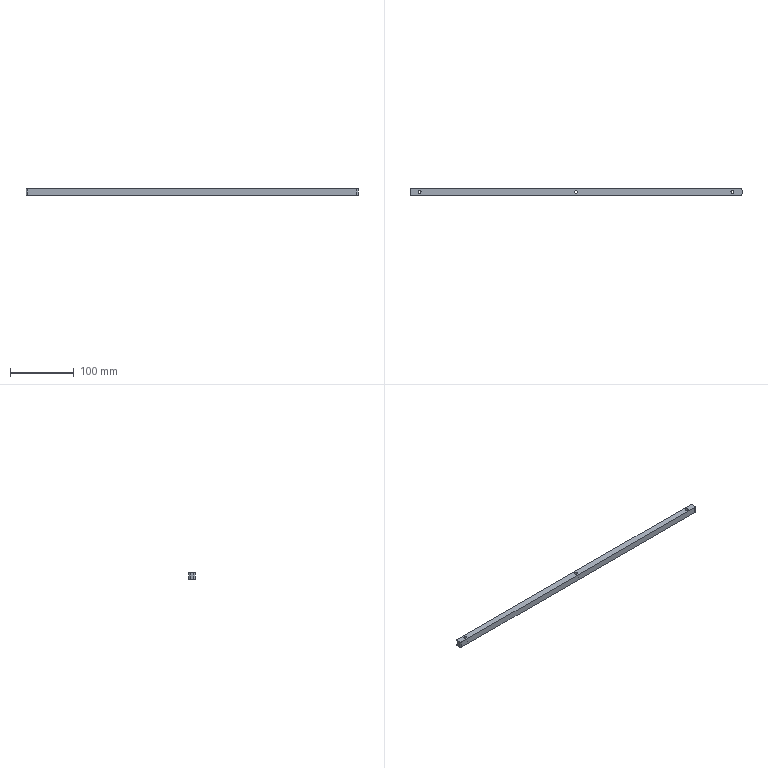Component | SolidWorks | SL010-RightStreamline-1-1_SL010-02047843SupportBar1-1-1 | 1 solid | 25 faces | box 520 x 10 x 10 mm | volume 51035 mm3 | cylinder 16 | plane 9 | commonest cylinder face diameters 8 x6 4.5 x6 4 x4 | material White POM
build123d program:
from build123d import *

# Parameters (mm, degrees)
SKETCH1_W                                       = 520
SKETCH1_H                                       = 10
BOSS_EXTRUDE1_DEPTH                             = 5
M4_HEX_SOCKET_HEAD_CAP_SCREW_CBORE1_D           = 4.5
M4_HEX_SOCKET_HEAD_CAP_SCREW_CBORE1_CBORE_D     = 8
M4_HEX_SOCKET_HEAD_CAP_SCREW_CBORE1_CBORE_DEPTH = 4.4
FILLET1_R                                       = 2


with BuildPart() as part:
    # Sketch1 → Boss-Extrude1 (new, symmetric)
    with BuildSketch(Plane.XY):
        Rectangle(SKETCH1_W, SKETCH1_H)
    extrude(amount=BOSS_EXTRUDE1_DEPTH, both=True)

    # M4 Hex Socket Head Cap Screw CBORE1 (through all)
    with Locations(Plane.XY.offset(5)):
        with Locations((-245, 0), (245, 0), (0, 0)):
            CounterBoreHole(M4_HEX_SOCKET_HEAD_CAP_SCREW_CBORE1_D / 2, M4_HEX_SOCKET_HEAD_CAP_SCREW_CBORE1_CBORE_D / 2, M4_HEX_SOCKET_HEAD_CAP_SCREW_CBORE1_CBORE_DEPTH)

    # Fillet1
    fillet1_edges = [part.edges().sort_by_distance(p)[0] for p in [
        (260, -5, 0),
        (-260, -5, 0),
        (-260, 5, 0),
        (260, 5, 0),
    ]]
    fillet(fillet1_edges, radius=FILLET1_R)


solid = part.part

# Placed as in the assembly
solid = solid.moved(Location((638.47, -116.404, -336.035), (180, 0, 0)))
STEP:
#1=COLOUR_RGB('',0.7922,0.8196,0.9333);
#2=FILL_AREA_STYLE_COLOUR('',#1);
#3=FILL_AREA_STYLE('',(#2));
#4=SURFACE_STYLE_FILL_AREA(#3);
#5=SURFACE_SIDE_STYLE('',(#4));
#6=SURFACE_STYLE_USAGE(.BOTH.,#5);
#7=PRESENTATION_STYLE_ASSIGNMENT((#6));
#8=CARTESIAN_POINT('',(34.94,-4.583,-13.253));
#9=VERTEX_POINT('',#8);
#10=CARTESIAN_POINT('',(34.625,-4.583,-13.253));
#11=VERTEX_POINT('',#10);
#12=CARTESIAN_POINT('',(34.782,-4.583,-13.253));
#13=DIRECTION('',(0.,-0.,-1.));
#14=DIRECTION('',(-1.,0.,0.));
#15=AXIS2_PLACEMENT_3D('',#12,#13,#14);
#16=CIRCLE('',#15,0.1575);
#17=EDGE_CURVE('',#9,#11,#16,.T.);
#18=ORIENTED_EDGE('',*,*,#17,.F.);
#19=CARTESIAN_POINT('',(34.94,-4.583,-13.427));
#20=VERTEX_POINT('',#19);
#21=CARTESIAN_POINT('',(34.94,-4.583,-13.427));
#22=DIRECTION('',(0.,-0.,-1.));
#23=VECTOR('',#22,39.37);
#24=LINE('',#21,#23);
#25=EDGE_CURVE('',#9,#20,#24,.T.);
#26=ORIENTED_EDGE('',*,*,#25,.T.);
#27=CARTESIAN_POINT('',(34.625,-4.583,-13.427));
#28=VERTEX_POINT('',#27);
#29=CARTESIAN_POINT('',(34.782,-4.583,-13.427));
#30=DIRECTION('',(0.,-0.,-1.));
#31=DIRECTION('',(-1.,0.,0.));
#32=AXIS2_PLACEMENT_3D('',#29,#30,#31);
#33=CIRCLE('',#32,0.1575);
#34=EDGE_CURVE('',#20,#28,#33,.T.);
#35=ORIENTED_EDGE('',*,*,#34,.T.);
#36=CARTESIAN_POINT('',(34.625,-4.583,-13.427));
#37=DIRECTION('',(0.,-0.,-1.));
#38=VECTOR('',#37,39.37);
#39=LINE('',#36,#38);
#40=EDGE_CURVE('',#11,#28,#39,.T.);
#41=ORIENTED_EDGE('',*,*,#40,.F.);
#42=EDGE_LOOP('',(#18,#26,#35,#41));
#43=FACE_OUTER_BOUND('',#42,.T.);
#44=CARTESIAN_POINT('',(34.782,-4.583,-13.427));
#45=DIRECTION('',(0.,-0.,-1.));
#46=DIRECTION('',(-1.,0.,0.));
#47=AXIS2_PLACEMENT_3D('',#44,#45,#46);
#48=CYLINDRICAL_SURFACE('',#47,0.1575);
#49=ADVANCED_FACE('',(#43),#48,.F.);
#50=CARTESIAN_POINT('',(34.871,-4.583,-13.033));
#51=VERTEX_POINT('',#50);
#52=CARTESIAN_POINT('',(34.694,-4.583,-13.033));
#53=VERTEX_POINT('',#52);
#54=CARTESIAN_POINT('',(34.782,-4.583,-13.033));
#55=DIRECTION('',(0.,-0.,-1.));
#56=DIRECTION('',(-1.,0.,0.));
#57=AXIS2_PLACEMENT_3D('',#54,#55,#56);
#58=CIRCLE('',#57,0.08858);
#59=EDGE_CURVE('',#51,#53,#58,.T.);
#60=ORIENTED_EDGE('',*,*,#59,.F.);
#61=CARTESIAN_POINT('',(34.871,-4.583,-13.253));
#62=VERTEX_POINT('',#61);
#63=CARTESIAN_POINT('',(34.871,-4.583,-13.427));
#64=DIRECTION('',(0.,-0.,-1.));
#65=VECTOR('',#64,39.37);
#66=LINE('',#63,#65);
#67=EDGE_CURVE('',#51,#62,#66,.T.);
#68=ORIENTED_EDGE('',*,*,#67,.T.);
#69=CARTESIAN_POINT('',(34.694,-4.583,-13.253));
#70=VERTEX_POINT('',#69);
#71=CARTESIAN_POINT('',(34.782,-4.583,-13.253));
#72=DIRECTION('',(0.,-0.,-1.));
#73=DIRECTION('',(-1.,0.,0.));
#74=AXIS2_PLACEMENT_3D('',#71,#72,#73);
#75=CIRCLE('',#74,0.08858);
#76=EDGE_CURVE('',#62,#70,#75,.T.);
#77=ORIENTED_EDGE('',*,*,#76,.T.);
#78=CARTESIAN_POINT('',(34.694,-4.583,-13.427));
#79=DIRECTION('',(0.,-0.,-1.));
#80=VECTOR('',#79,39.37);
#81=LINE('',#78,#80);
#82=EDGE_CURVE('',#53,#70,#81,.T.);
#83=ORIENTED_EDGE('',*,*,#82,.F.);
#84=EDGE_LOOP('',(#60,#68,#77,#83));
#85=FACE_OUTER_BOUND('',#84,.T.);
#86=CARTESIAN_POINT('',(34.782,-4.583,-13.427));
#87=DIRECTION('',(0.,-0.,-1.));
#88=DIRECTION('',(-1.,0.,0.));
#89=AXIS2_PLACEMENT_3D('',#86,#87,#88);
#90=CYLINDRICAL_SURFACE('',#89,0.08858);
#91=ADVANCED_FACE('',(#85),#90,.F.);
#92=CARTESIAN_POINT('',(15.648,-4.583,-13.253));
#93=VERTEX_POINT('',#92);
#94=CARTESIAN_POINT('',(15.333,-4.583,-13.253));
#95=VERTEX_POINT('',#94);
#96=CARTESIAN_POINT('',(15.491,-4.583,-13.253));
#97=DIRECTION('',(0.,-0.,-1.));
#98=DIRECTION('',(-1.,0.,0.));
#99=AXIS2_PLACEMENT_3D('',#96,#97,#98);
#100=CIRCLE('',#99,0.1575);
#101=EDGE_CURVE('',#93,#95,#100,.T.);
#102=ORIENTED_EDGE('',*,*,#101,.F.);
#103=CARTESIAN_POINT('',(15.648,-4.583,-13.427));
#104=VERTEX_POINT('',#103);
#105=CARTESIAN_POINT('',(15.648,-4.583,-13.427));
#106=DIRECTION('',(0.,-0.,-1.));
#107=VECTOR('',#106,39.37);
#108=LINE('',#105,#107);
#109=EDGE_CURVE('',#93,#104,#108,.T.);
#110=ORIENTED_EDGE('',*,*,#109,.T.);
#111=CARTESIAN_POINT('',(15.333,-4.583,-13.427));
#112=VERTEX_POINT('',#111);
#113=CARTESIAN_POINT('',(15.491,-4.583,-13.427));
#114=DIRECTION('',(0.,-0.,-1.));
#115=DIRECTION('',(-1.,0.,0.));
#116=AXIS2_PLACEMENT_3D('',#113,#114,#115);
#117=CIRCLE('',#116,0.1575);
#118=EDGE_CURVE('',#104,#112,#117,.T.);
#119=ORIENTED_EDGE('',*,*,#118,.T.);
#120=CARTESIAN_POINT('',(15.333,-4.583,-13.427));
#121=DIRECTION('',(0.,-0.,-1.));
#122=VECTOR('',#121,39.37);
#123=LINE('',#120,#122);
#124=EDGE_CURVE('',#95,#112,#123,.T.);
#125=ORIENTED_EDGE('',*,*,#124,.F.);
#126=EDGE_LOOP('',(#102,#110,#119,#125));
#127=FACE_OUTER_BOUND('',#126,.T.);
#128=CARTESIAN_POINT('',(15.491,-4.583,-13.427));
#129=DIRECTION('',(0.,-0.,-1.));
#130=DIRECTION('',(-1.,0.,0.));
#131=AXIS2_PLACEMENT_3D('',#128,#129,#130);
#132=CYLINDRICAL_SURFACE('',#131,0.1575);
#133=ADVANCED_FACE('',(#127),#132,.F.);
#134=CARTESIAN_POINT('',(15.58,-4.583,-13.033));
#135=VERTEX_POINT('',#134);
#136=CARTESIAN_POINT('',(15.402,-4.583,-13.033));
#137=VERTEX_POINT('',#136);
#138=CARTESIAN_POINT('',(15.491,-4.583,-13.033));
#139=DIRECTION('',(0.,-0.,-1.));
#140=DIRECTION('',(-1.,0.,0.));
#141=AXIS2_PLACEMENT_3D('',#138,#139,#140);
#142=CIRCLE('',#141,0.08858);
#143=EDGE_CURVE('',#135,#137,#142,.T.);
#144=ORIENTED_EDGE('',*,*,#143,.F.);
#145=CARTESIAN_POINT('',(15.58,-4.583,-13.253));
#146=VERTEX_POINT('',#145);
#147=CARTESIAN_POINT('',(15.58,-4.583,-13.427));
#148=DIRECTION('',(0.,-0.,-1.));
#149=VECTOR('',#148,39.37);
#150=LINE('',#147,#149);
#151=EDGE_CURVE('',#135,#146,#150,.T.);
#152=ORIENTED_EDGE('',*,*,#151,.T.);
#153=CARTESIAN_POINT('',(15.402,-4.583,-13.253));
#154=VERTEX_POINT('',#153);
#155=CARTESIAN_POINT('',(15.491,-4.583,-13.253));
#156=DIRECTION('',(0.,-0.,-1.));
#157=DIRECTION('',(-1.,0.,0.));
#158=AXIS2_PLACEMENT_3D('',#155,#156,#157);
#159=CIRCLE('',#158,0.08858);
#160=EDGE_CURVE('',#146,#154,#159,.T.);
#161=ORIENTED_EDGE('',*,*,#160,.T.);
#162=CARTESIAN_POINT('',(15.402,-4.583,-13.427));
#163=DIRECTION('',(0.,-0.,-1.));
#164=VECTOR('',#163,39.37);
#165=LINE('',#162,#164);
#166=EDGE_CURVE('',#137,#154,#165,.T.);
#167=ORIENTED_EDGE('',*,*,#166,.F.);
#168=EDGE_LOOP('',(#144,#152,#161,#167));
#169=FACE_OUTER_BOUND('',#168,.T.);
#170=CARTESIAN_POINT('',(15.491,-4.583,-13.427));
#171=DIRECTION('',(0.,-0.,-1.));
#172=DIRECTION('',(-1.,0.,0.));
#173=AXIS2_PLACEMENT_3D('',#170,#171,#172);
#174=CYLINDRICAL_SURFACE('',#173,0.08858);
#175=ADVANCED_FACE('',(#169),#174,.F.);
#176=CARTESIAN_POINT('',(25.294,-4.583,-13.253));
#177=VERTEX_POINT('',#176);
#178=CARTESIAN_POINT('',(24.979,-4.583,-13.253));
#179=VERTEX_POINT('',#178);
#180=CARTESIAN_POINT('',(25.137,-4.583,-13.253));
#181=DIRECTION('',(0.,-0.,-1.));
#182=DIRECTION('',(-1.,0.,0.));
#183=AXIS2_PLACEMENT_3D('',#180,#181,#182);
#184=CIRCLE('',#183,0.1575);
#185=EDGE_CURVE('',#177,#179,#184,.T.);
#186=ORIENTED_EDGE('',*,*,#185,.F.);
#187=CARTESIAN_POINT('',(25.294,-4.583,-13.427));
#188=VERTEX_POINT('',#187);
#189=CARTESIAN_POINT('',(25.294,-4.583,-13.427));
#190=DIRECTION('',(0.,-0.,-1.));
#191=VECTOR('',#190,39.37);
#192=LINE('',#189,#191);
#193=EDGE_CURVE('',#177,#188,#192,.T.);
#194=ORIENTED_EDGE('',*,*,#193,.T.);
#195=CARTESIAN_POINT('',(24.979,-4.583,-13.427));
#196=VERTEX_POINT('',#195);
#197=CARTESIAN_POINT('',(25.137,-4.583,-13.427));
#198=DIRECTION('',(0.,-0.,-1.));
#199=DIRECTION('',(-1.,0.,0.));
#200=AXIS2_PLACEMENT_3D('',#197,#198,#199);
#201=CIRCLE('',#200,0.1575);
#202=EDGE_CURVE('',#188,#196,#201,.T.);
#203=ORIENTED_EDGE('',*,*,#202,.T.);
#204=CARTESIAN_POINT('',(24.979,-4.583,-13.427));
#205=DIRECTION('',(0.,-0.,-1.));
#206=VECTOR('',#205,39.37);
#207=LINE('',#204,#206);
#208=EDGE_CURVE('',#179,#196,#207,.T.);
#209=ORIENTED_EDGE('',*,*,#208,.F.);
#210=EDGE_LOOP('',(#186,#194,#203,#209));
#211=FACE_OUTER_BOUND('',#210,.T.);
#212=CARTESIAN_POINT('',(25.137,-4.583,-13.427));
#213=DIRECTION('',(0.,-0.,-1.));
#214=DIRECTION('',(-1.,0.,0.));
#215=AXIS2_PLACEMENT_3D('',#212,#213,#214);
#216=CYLINDRICAL_SURFACE('',#215,0.1575);
#217=ADVANCED_FACE('',(#211),#216,.F.);
#218=CARTESIAN_POINT('',(25.225,-4.583,-13.033));
#219=VERTEX_POINT('',#218);
#220=CARTESIAN_POINT('',(25.048,-4.583,-13.033));
#221=VERTEX_POINT('',#220);
#222=CARTESIAN_POINT('',(25.137,-4.583,-13.033));
#223=DIRECTION('',(0.,-0.,-1.));
#224=DIRECTION('',(-1.,0.,0.));
#225=AXIS2_PLACEMENT_3D('',#222,#223,#224);
#226=CIRCLE('',#225,0.08858);
#227=EDGE_CURVE('',#219,#221,#226,.T.);
#228=ORIENTED_EDGE('',*,*,#227,.F.);
#229=CARTESIAN_POINT('',(25.225,-4.583,-13.253));
#230=VERTEX_POINT('',#229);
#231=CARTESIAN_POINT('',(25.225,-4.583,-13.427));
#232=DIRECTION('',(0.,-0.,-1.));
#233=VECTOR('',#232,39.37);
#234=LINE('',#231,#233);
#235=EDGE_CURVE('',#219,#230,#234,.T.);
#236=ORIENTED_EDGE('',*,*,#235,.T.);
#237=CARTESIAN_POINT('',(25.048,-4.583,-13.253));
#238=VERTEX_POINT('',#237);
#239=CARTESIAN_POINT('',(25.137,-4.583,-13.253));
#240=DIRECTION('',(0.,-0.,-1.));
#241=DIRECTION('',(-1.,0.,0.));
#242=AXIS2_PLACEMENT_3D('',#239,#240,#241);
#243=CIRCLE('',#242,0.08858);
#244=EDGE_CURVE('',#230,#238,#243,.T.);
#245=ORIENTED_EDGE('',*,*,#244,.T.);
#246=CARTESIAN_POINT('',(25.048,-4.583,-13.427));
#247=DIRECTION('',(0.,-0.,-1.));
#248=VECTOR('',#247,39.37);
#249=LINE('',#246,#248);
#250=EDGE_CURVE('',#221,#238,#249,.T.);
#251=ORIENTED_EDGE('',*,*,#250,.F.);
#252=EDGE_LOOP('',(#228,#236,#245,#251));
#253=FACE_OUTER_BOUND('',#252,.T.);
#254=CARTESIAN_POINT('',(25.137,-4.583,-13.427));
#255=DIRECTION('',(0.,-0.,-1.));
#256=DIRECTION('',(-1.,0.,0.));
#257=AXIS2_PLACEMENT_3D('',#254,#255,#256);
#258=CYLINDRICAL_SURFACE('',#257,0.08858);
#259=ADVANCED_FACE('',(#253),#258,.F.);
#260=CARTESIAN_POINT('',(14.9,-4.701,-13.427));
#261=VERTEX_POINT('',#260);
#262=CARTESIAN_POINT('',(14.9,-4.465,-13.427));
#263=VERTEX_POINT('',#262);
#264=CARTESIAN_POINT('',(14.9,-4.386,-13.427));
#265=DIRECTION('',(0.,1.,-0.));
#266=VECTOR('',#265,39.37);
#267=LINE('',#264,#266);
#268=EDGE_CURVE('',#261,#263,#267,.T.);
#269=ORIENTED_EDGE('',*,*,#268,.F.);
#270=CARTESIAN_POINT('',(14.9,-4.701,-13.033));
#271=VERTEX_POINT('',#270);
#272=CARTESIAN_POINT('',(14.9,-4.701,-13.427));
#273=DIRECTION('',(-0.,0.,1.));
#274=VECTOR('',#273,39.37);
#275=LINE('',#272,#274);
#276=EDGE_CURVE('',#261,#271,#275,.T.);
#277=ORIENTED_EDGE('',*,*,#276,.T.);
#278=CARTESIAN_POINT('',(14.9,-4.465,-13.033));
#279=VERTEX_POINT('',#278);
#280=CARTESIAN_POINT('',(14.9,-4.386,-13.033));
#281=DIRECTION('',(0.,1.,-0.));
#282=VECTOR('',#281,39.37);
#283=LINE('',#280,#282);
#284=EDGE_CURVE('',#271,#279,#283,.T.);
#285=ORIENTED_EDGE('',*,*,#284,.T.);
#286=CARTESIAN_POINT('',(14.9,-4.465,-13.427));
#287=DIRECTION('',(0.,-0.,-1.));
#288=VECTOR('',#287,39.37);
#289=LINE('',#286,#288);
#290=EDGE_CURVE('',#279,#263,#289,.T.);
#291=ORIENTED_EDGE('',*,*,#290,.T.);
#292=EDGE_LOOP('',(#269,#277,#285,#291));
#293=FACE_OUTER_BOUND('',#292,.T.);
#294=CARTESIAN_POINT('',(14.9,-4.386,-13.427));
#295=DIRECTION('',(1.,-0.,0.));
#296=DIRECTION('',(0.,-0.,-1.));
#297=AXIS2_PLACEMENT_3D('',#294,#295,#296);
#298=PLANE('',#297);
#299=ADVANCED_FACE('',(#293),#298,.F.);
#300=CARTESIAN_POINT('',(14.979,-4.386,-13.427));
#301=VERTEX_POINT('',#300);
#302=CARTESIAN_POINT('',(35.294,-4.386,-13.427));
#303=VERTEX_POINT('',#302);
#304=CARTESIAN_POINT('',(35.373,-4.386,-13.427));
#305=DIRECTION('',(1.,-0.,0.));
#306=VECTOR('',#305,39.37);
#307=LINE('',#304,#306);
#308=EDGE_CURVE('',#301,#303,#307,.T.);
#309=ORIENTED_EDGE('',*,*,#308,.F.);
#310=CARTESIAN_POINT('',(14.979,-4.386,-13.033));
#311=VERTEX_POINT('',#310);
#312=CARTESIAN_POINT('',(14.979,-4.386,-13.427));
#313=DIRECTION('',(-0.,0.,1.));
#314=VECTOR('',#313,39.37);
#315=LINE('',#312,#314);
#316=EDGE_CURVE('',#301,#311,#315,.T.);
#317=ORIENTED_EDGE('',*,*,#316,.T.);
#318=CARTESIAN_POINT('',(35.294,-4.386,-13.033));
#319=VERTEX_POINT('',#318);
#320=CARTESIAN_POINT('',(35.373,-4.386,-13.033));
#321=DIRECTION('',(1.,-0.,0.));
#322=VECTOR('',#321,39.37);
#323=LINE('',#320,#322);
#324=EDGE_CURVE('',#311,#319,#323,.T.);
#325=ORIENTED_EDGE('',*,*,#324,.T.);
#326=CARTESIAN_POINT('',(35.294,-4.386,-13.427));
#327=DIRECTION('',(0.,-0.,-1.));
#328=VECTOR('',#327,39.37);
#329=LINE('',#326,#328);
#330=EDGE_CURVE('',#319,#303,#329,.T.);
#331=ORIENTED_EDGE('',*,*,#330,.T.);
#332=EDGE_LOOP('',(#309,#317,#325,#331));
#333=FACE_OUTER_BOUND('',#332,.T.);
#334=CARTESIAN_POINT('',(35.373,-4.386,-13.427));
#335=DIRECTION('',(-0.,-1.,0.));
#336=DIRECTION('',(-0.,0.,1.));
#337=AXIS2_PLACEMENT_3D('',#334,#335,#336);
#338=PLANE('',#337);
#339=ADVANCED_FACE('',(#333),#338,.F.);
#340=CARTESIAN_POINT('',(35.373,-4.465,-13.033));
#341=VERTEX_POINT('',#340);
#342=CARTESIAN_POINT('',(35.373,-4.701,-13.033));
#343=VERTEX_POINT('',#342);
#344=CARTESIAN_POINT('',(35.373,-4.386,-13.033));
#345=DIRECTION('',(-0.,-1.,0.));
#346=VECTOR('',#345,39.37);
#347=LINE('',#344,#346);
#348=EDGE_CURVE('',#341,#343,#347,.T.);
#349=ORIENTED_EDGE('',*,*,#348,.T.);
#350=CARTESIAN_POINT('',(35.373,-4.701,-13.427));
#351=VERTEX_POINT('',#350);
#352=CARTESIAN_POINT('',(35.373,-4.701,-13.427));
#353=DIRECTION('',(0.,-0.,-1.));
#354=VECTOR('',#353,39.37);
#355=LINE('',#352,#354);
#356=EDGE_CURVE('',#343,#351,#355,.T.);
#357=ORIENTED_EDGE('',*,*,#356,.T.);
#358=CARTESIAN_POINT('',(35.373,-4.465,-13.427));
#359=VERTEX_POINT('',#358);
#360=CARTESIAN_POINT('',(35.373,-4.386,-13.427));
#361=DIRECTION('',(-0.,-1.,0.));
#362=VECTOR('',#361,39.37);
#363=LINE('',#360,#362);
#364=EDGE_CURVE('',#359,#351,#363,.T.);
#365=ORIENTED_EDGE('',*,*,#364,.F.);
#366=CARTESIAN_POINT('',(35.373,-4.465,-13.427));
#367=DIRECTION('',(-0.,0.,1.));
#368=VECTOR('',#367,39.37);
#369=LINE('',#366,#368);
#370=EDGE_CURVE('',#359,#341,#369,.T.);
#371=ORIENTED_EDGE('',*,*,#370,.T.);
#372=EDGE_LOOP('',(#349,#357,#365,#371));
#373=FACE_OUTER_BOUND('',#372,.T.);
#374=CARTESIAN_POINT('',(35.373,-4.386,-13.427));
#375=DIRECTION('',(-1.,0.,-0.));
#376=DIRECTION('',(-0.,0.,1.));
#377=AXIS2_PLACEMENT_3D('',#374,#375,#376);
#378=PLANE('',#377);
#379=ADVANCED_FACE('',(#373),#378,.F.);
#380=CARTESIAN_POINT('',(35.294,-4.78,-13.033));
#381=VERTEX_POINT('',#380);
#382=CARTESIAN_POINT('',(14.979,-4.78,-13.033));
#383=VERTEX_POINT('',#382);
#384=CARTESIAN_POINT('',(35.373,-4.78,-13.033));
#385=DIRECTION('',(-1.,0.,-0.));
#386=VECTOR('',#385,39.37);
#387=LINE('',#384,#386);
#388=EDGE_CURVE('',#381,#383,#387,.T.);
#389=ORIENTED_EDGE('',*,*,#388,.T.);
#390=CARTESIAN_POINT('',(14.979,-4.78,-13.427));
#391=VERTEX_POINT('',#390);
#392=CARTESIAN_POINT('',(14.979,-4.78,-13.427));
#393=DIRECTION('',(0.,-0.,-1.));
#394=VECTOR('',#393,39.37);
#395=LINE('',#392,#394);
#396=EDGE_CURVE('',#383,#391,#395,.T.);
#397=ORIENTED_EDGE('',*,*,#396,.T.);
#398=CARTESIAN_POINT('',(35.294,-4.78,-13.427));
#399=VERTEX_POINT('',#398);
#400=CARTESIAN_POINT('',(35.373,-4.78,-13.427));
#401=DIRECTION('',(-1.,0.,-0.));
#402=VECTOR('',#401,39.37);
#403=LINE('',#400,#402);
#404=EDGE_CURVE('',#399,#391,#403,.T.);
#405=ORIENTED_EDGE('',*,*,#404,.F.);
#406=CARTESIAN_POINT('',(35.294,-4.78,-13.427));
#407=DIRECTION('',(-0.,0.,1.));
#408=VECTOR('',#407,39.37);
#409=LINE('',#406,#408);
#410=EDGE_CURVE('',#399,#381,#409,.T.);
#411=ORIENTED_EDGE('',*,*,#410,.T.);
#412=EDGE_LOOP('',(#389,#397,#405,#411));
#413=FACE_OUTER_BOUND('',#412,.T.);
#414=CARTESIAN_POINT('',(35.373,-4.78,-13.427));
#415=DIRECTION('',(0.,1.,-0.));
#416=DIRECTION('',(0.,-0.,-1.));
#417=AXIS2_PLACEMENT_3D('',#414,#415,#416);
#418=PLANE('',#417);
#419=ADVANCED_FACE('',(#413),#418,.F.);
#420=CARTESIAN_POINT('',(34.782,-4.583,-13.427));
#421=DIRECTION('',(0.,-0.,-1.));
#422=DIRECTION('',(-1.,0.,0.));
#423=AXIS2_PLACEMENT_3D('',#420,#421,#422);
#424=CIRCLE('',#423,0.1575);
#425=EDGE_CURVE('',#28,#20,#424,.T.);
#426=ORIENTED_EDGE('',*,*,#425,.F.);
#427=ORIENTED_EDGE('',*,*,#34,.F.);
#428=EDGE_LOOP('',(#426,#427));
#429=FACE_BOUND('',#428,.T.);
#430=CARTESIAN_POINT('',(15.491,-4.583,-13.427));
#431=DIRECTION('',(0.,-0.,-1.));
#432=DIRECTION('',(-1.,0.,0.));
#433=AXIS2_PLACEMENT_3D('',#430,#431,#432);
#434=CIRCLE('',#433,0.1575);
#435=EDGE_CURVE('',#112,#104,#434,.T.);
#436=ORIENTED_EDGE('',*,*,#435,.F.);
#437=ORIENTED_EDGE('',*,*,#118,.F.);
#438=EDGE_LOOP('',(#436,#437));
#439=FACE_BOUND('',#438,.T.);
#440=CARTESIAN_POINT('',(25.137,-4.583,-13.427));
#441=DIRECTION('',(0.,-0.,-1.));
#442=DIRECTION('',(-1.,0.,0.));
#443=AXIS2_PLACEMENT_3D('',#440,#441,#442);
#444=CIRCLE('',#443,0.1575);
#445=EDGE_CURVE('',#196,#188,#444,.T.);
#446=ORIENTED_EDGE('',*,*,#445,.F.);
#447=ORIENTED_EDGE('',*,*,#202,.F.);
#448=EDGE_LOOP('',(#446,#447));
#449=FACE_BOUND('',#448,.T.);
#450=ORIENTED_EDGE('',*,*,#404,.T.);
#451=CARTESIAN_POINT('',(14.979,-4.701,-13.427));
#452=DIRECTION('',(0.,-0.,-1.));
#453=DIRECTION('',(-1.,0.,0.));
#454=AXIS2_PLACEMENT_3D('',#451,#452,#453);
#455=CIRCLE('',#454,0.07874);
#456=EDGE_CURVE('',#391,#261,#455,.T.);
#457=ORIENTED_EDGE('',*,*,#456,.T.);
#458=ORIENTED_EDGE('',*,*,#268,.T.);
#459=CARTESIAN_POINT('',(14.979,-4.465,-13.427));
#460=DIRECTION('',(0.,-0.,-1.));
#461=DIRECTION('',(-1.,0.,0.));
#462=AXIS2_PLACEMENT_3D('',#459,#460,#461);
#463=CIRCLE('',#462,0.07874);
#464=EDGE_CURVE('',#263,#301,#463,.T.);
#465=ORIENTED_EDGE('',*,*,#464,.T.);
#466=ORIENTED_EDGE('',*,*,#308,.T.);
#467=CARTESIAN_POINT('',(35.294,-4.465,-13.427));
#468=DIRECTION('',(0.,-0.,-1.));
#469=DIRECTION('',(-1.,0.,0.));
#470=AXIS2_PLACEMENT_3D('',#467,#468,#469);
#471=CIRCLE('',#470,0.07874);
#472=EDGE_CURVE('',#303,#359,#471,.T.);
#473=ORIENTED_EDGE('',*,*,#472,.T.);
#474=ORIENTED_EDGE('',*,*,#364,.T.);
#475=CARTESIAN_POINT('',(35.294,-4.701,-13.427));
#476=DIRECTION('',(0.,-0.,-1.));
#477=DIRECTION('',(-1.,0.,0.));
#478=AXIS2_PLACEMENT_3D('',#475,#476,#477);
#479=CIRCLE('',#478,0.07874);
#480=EDGE_CURVE('',#351,#399,#479,.T.);
#481=ORIENTED_EDGE('',*,*,#480,.T.);
#482=EDGE_LOOP('',(#450,#457,#458,#465,#466,#473,#474,#481));
#483=FACE_OUTER_BOUND('',#482,.T.);
#484=CARTESIAN_POINT('',(25.137,-4.583,-13.427));
#485=DIRECTION('',(0.,-0.,-1.));
#486=DIRECTION('',(-1.,0.,-0.));
#487=AXIS2_PLACEMENT_3D('',#484,#485,#486);
#488=PLANE('',#487);
#489=ADVANCED_FACE('',(#429,#439,#449,#483),#488,.T.);
#490=CARTESIAN_POINT('',(34.782,-4.583,-13.033));
#491=DIRECTION('',(0.,-0.,-1.));
#492=DIRECTION('',(-1.,0.,0.));
#493=AXIS2_PLACEMENT_3D('',#490,#491,#492);
#494=CIRCLE('',#493,0.08858);
#495=EDGE_CURVE('',#53,#51,#494,.T.);
#496=ORIENTED_EDGE('',*,*,#495,.T.);
#497=ORIENTED_EDGE('',*,*,#59,.T.);
#498=EDGE_LOOP('',(#496,#497));
#499=FACE_BOUND('',#498,.T.);
#500=CARTESIAN_POINT('',(15.491,-4.583,-13.033));
#501=DIRECTION('',(0.,-0.,-1.));
#502=DIRECTION('',(-1.,0.,0.));
#503=AXIS2_PLACEMENT_3D('',#500,#501,#502);
#504=CIRCLE('',#503,0.08858);
#505=EDGE_CURVE('',#137,#135,#504,.T.);
#506=ORIENTED_EDGE('',*,*,#505,.T.);
#507=ORIENTED_EDGE('',*,*,#143,.T.);
#508=EDGE_LOOP('',(#506,#507));
#509=FACE_BOUND('',#508,.T.);
#510=CARTESIAN_POINT('',(25.137,-4.583,-13.033));
#511=DIRECTION('',(0.,-0.,-1.));
#512=DIRECTION('',(-1.,0.,0.));
#513=AXIS2_PLACEMENT_3D('',#510,#511,#512);
#514=CIRCLE('',#513,0.08858);
#515=EDGE_CURVE('',#221,#219,#514,.T.);
#516=ORIENTED_EDGE('',*,*,#515,.T.);
#517=ORIENTED_EDGE('',*,*,#227,.T.);
#518=EDGE_LOOP('',(#516,#517));
#519=FACE_BOUND('',#518,.T.);
#520=ORIENTED_EDGE('',*,*,#284,.F.);
#521=CARTESIAN_POINT('',(14.979,-4.701,-13.033));
#522=DIRECTION('',(-0.,0.,1.));
#523=DIRECTION('',(-1.,0.,0.));
#524=AXIS2_PLACEMENT_3D('',#521,#522,#523);
#525=CIRCLE('',#524,0.07874);
#526=EDGE_CURVE('',#271,#383,#525,.T.);
#527=ORIENTED_EDGE('',*,*,#526,.T.);
#528=ORIENTED_EDGE('',*,*,#388,.F.);
#529=CARTESIAN_POINT('',(35.294,-4.701,-13.033));
#530=DIRECTION('',(-0.,0.,1.));
#531=DIRECTION('',(-1.,0.,0.));
#532=AXIS2_PLACEMENT_3D('',#529,#530,#531);
#533=CIRCLE('',#532,0.07874);
#534=EDGE_CURVE('',#381,#343,#533,.T.);
#535=ORIENTED_EDGE('',*,*,#534,.T.);
#536=ORIENTED_EDGE('',*,*,#348,.F.);
#537=CARTESIAN_POINT('',(35.294,-4.465,-13.033));
#538=DIRECTION('',(-0.,0.,1.));
#539=DIRECTION('',(-1.,0.,0.));
#540=AXIS2_PLACEMENT_3D('',#537,#538,#539);
#541=CIRCLE('',#540,0.07874);
#542=EDGE_CURVE('',#341,#319,#541,.T.);
#543=ORIENTED_EDGE('',*,*,#542,.T.);
#544=ORIENTED_EDGE('',*,*,#324,.F.);
#545=CARTESIAN_POINT('',(14.979,-4.465,-13.033));
#546=DIRECTION('',(-0.,0.,1.));
#547=DIRECTION('',(-1.,0.,0.));
#548=AXIS2_PLACEMENT_3D('',#545,#546,#547);
#549=CIRCLE('',#548,0.07874);
#550=EDGE_CURVE('',#311,#279,#549,.T.);
#551=ORIENTED_EDGE('',*,*,#550,.T.);
#552=EDGE_LOOP('',(#520,#527,#528,#535,#536,#543,#544,#551));
#553=FACE_OUTER_BOUND('',#552,.T.);
#554=CARTESIAN_POINT('',(25.137,-4.583,-13.033));
#555=DIRECTION('',(0.,-0.,-1.));
#556=DIRECTION('',(-1.,0.,-0.));
#557=AXIS2_PLACEMENT_3D('',#554,#555,#556);
#558=PLANE('',#557);
#559=ADVANCED_FACE('',(#499,#509,#519,#553),#558,.F.);
#560=ORIENTED_EDGE('',*,*,#235,.F.);
#561=ORIENTED_EDGE('',*,*,#515,.F.);
#562=ORIENTED_EDGE('',*,*,#250,.T.);
#563=CARTESIAN_POINT('',(25.137,-4.583,-13.253));
#564=DIRECTION('',(0.,-0.,-1.));
#565=DIRECTION('',(-1.,0.,0.));
#566=AXIS2_PLACEMENT_3D('',#563,#564,#565);
#567=CIRCLE('',#566,0.08858);
#568=EDGE_CURVE('',#238,#230,#567,.T.);
#569=ORIENTED_EDGE('',*,*,#568,.T.);
#570=EDGE_LOOP('',(#560,#561,#562,#569));
#571=FACE_OUTER_BOUND('',#570,.T.);
#572=CARTESIAN_POINT('',(25.137,-4.583,-13.427));
#573=DIRECTION('',(0.,-0.,-1.));
#574=DIRECTION('',(-1.,0.,0.));
#575=AXIS2_PLACEMENT_3D('',#572,#573,#574);
#576=CYLINDRICAL_SURFACE('',#575,0.08858);
#577=ADVANCED_FACE('',(#571),#576,.F.);
#578=ORIENTED_EDGE('',*,*,#568,.F.);
#579=ORIENTED_EDGE('',*,*,#244,.F.);
#580=EDGE_LOOP('',(#578,#579));
#581=FACE_BOUND('',#580,.T.);
#582=CARTESIAN_POINT('',(25.137,-4.583,-13.253));
#583=DIRECTION('',(0.,-0.,-1.));
#584=DIRECTION('',(-1.,0.,0.));
#585=AXIS2_PLACEMENT_3D('',#582,#583,#584);
#586=CIRCLE('',#585,0.1575);
#587=EDGE_CURVE('',#179,#177,#586,.T.);
#588=ORIENTED_EDGE('',*,*,#587,.T.);
#589=ORIENTED_EDGE('',*,*,#185,.T.);
#590=EDGE_LOOP('',(#588,#589));
#591=FACE_OUTER_BOUND('',#590,.T.);
#592=CARTESIAN_POINT('',(25.048,-4.583,-13.253));
#593=DIRECTION('',(-0.,0.,1.));
#594=DIRECTION('',(1.,-0.,0.));
#595=AXIS2_PLACEMENT_3D('',#592,#593,#594);
#596=PLANE('',#595);
#597=ADVANCED_FACE('',(#581,#591),#596,.F.);
#598=ORIENTED_EDGE('',*,*,#193,.F.);
#599=ORIENTED_EDGE('',*,*,#587,.F.);
#600=ORIENTED_EDGE('',*,*,#208,.T.);
#601=ORIENTED_EDGE('',*,*,#445,.T.);
#602=EDGE_LOOP('',(#598,#599,#600,#601));
#603=FACE_OUTER_BOUND('',#602,.T.);
#604=CARTESIAN_POINT('',(25.137,-4.583,-13.427));
#605=DIRECTION('',(0.,-0.,-1.));
#606=DIRECTION('',(-1.,0.,0.));
#607=AXIS2_PLACEMENT_3D('',#604,#605,#606);
#608=CYLINDRICAL_SURFACE('',#607,0.1575);
#609=ADVANCED_FACE('',(#603),#608,.F.);
#610=ORIENTED_EDGE('',*,*,#151,.F.);
#611=ORIENTED_EDGE('',*,*,#505,.F.);
#612=ORIENTED_EDGE('',*,*,#166,.T.);
#613=CARTESIAN_POINT('',(15.491,-4.583,-13.253));
#614=DIRECTION('',(0.,-0.,-1.));
#615=DIRECTION('',(-1.,0.,0.));
#616=AXIS2_PLACEMENT_3D('',#613,#614,#615);
#617=CIRCLE('',#616,0.08858);
#618=EDGE_CURVE('',#154,#146,#617,.T.);
#619=ORIENTED_EDGE('',*,*,#618,.T.);
#620=EDGE_LOOP('',(#610,#611,#612,#619));
#621=FACE_OUTER_BOUND('',#620,.T.);
#622=CARTESIAN_POINT('',(15.491,-4.583,-13.427));
#623=DIRECTION('',(0.,-0.,-1.));
#624=DIRECTION('',(-1.,0.,0.));
#625=AXIS2_PLACEMENT_3D('',#622,#623,#624);
#626=CYLINDRICAL_SURFACE('',#625,0.08858);
#627=ADVANCED_FACE('',(#621),#626,.F.);
#628=ORIENTED_EDGE('',*,*,#618,.F.);
#629=ORIENTED_EDGE('',*,*,#160,.F.);
#630=EDGE_LOOP('',(#628,#629));
#631=FACE_BOUND('',#630,.T.);
#632=CARTESIAN_POINT('',(15.491,-4.583,-13.253));
#633=DIRECTION('',(0.,-0.,-1.));
#634=DIRECTION('',(-1.,0.,0.));
#635=AXIS2_PLACEMENT_3D('',#632,#633,#634);
#636=CIRCLE('',#635,0.1575);
#637=EDGE_CURVE('',#95,#93,#636,.T.);
#638=ORIENTED_EDGE('',*,*,#637,.T.);
#639=ORIENTED_EDGE('',*,*,#101,.T.);
#640=EDGE_LOOP('',(#638,#639));
#641=FACE_OUTER_BOUND('',#640,.T.);
#642=CARTESIAN_POINT('',(15.402,-4.583,-13.253));
#643=DIRECTION('',(-0.,0.,1.));
#644=DIRECTION('',(1.,-0.,0.));
#645=AXIS2_PLACEMENT_3D('',#642,#643,#644);
#646=PLANE('',#645);
#647=ADVANCED_FACE('',(#631,#641),#646,.F.);
#648=ORIENTED_EDGE('',*,*,#109,.F.);
#649=ORIENTED_EDGE('',*,*,#637,.F.);
#650=ORIENTED_EDGE('',*,*,#124,.T.);
#651=ORIENTED_EDGE('',*,*,#435,.T.);
#652=EDGE_LOOP('',(#648,#649,#650,#651));
#653=FACE_OUTER_BOUND('',#652,.T.);
#654=CARTESIAN_POINT('',(15.491,-4.583,-13.427));
#655=DIRECTION('',(0.,-0.,-1.));
#656=DIRECTION('',(-1.,0.,0.));
#657=AXIS2_PLACEMENT_3D('',#654,#655,#656);
#658=CYLINDRICAL_SURFACE('',#657,0.1575);
#659=ADVANCED_FACE('',(#653),#658,.F.);
#660=ORIENTED_EDGE('',*,*,#67,.F.);
#661=ORIENTED_EDGE('',*,*,#495,.F.);
#662=ORIENTED_EDGE('',*,*,#82,.T.);
#663=CARTESIAN_POINT('',(34.782,-4.583,-13.253));
#664=DIRECTION('',(0.,-0.,-1.));
#665=DIRECTION('',(-1.,0.,0.));
#666=AXIS2_PLACEMENT_3D('',#663,#664,#665);
#667=CIRCLE('',#666,0.08858);
#668=EDGE_CURVE('',#70,#62,#667,.T.);
#669=ORIENTED_EDGE('',*,*,#668,.T.);
#670=EDGE_LOOP('',(#660,#661,#662,#669));
#671=FACE_OUTER_BOUND('',#670,.T.);
#672=CARTESIAN_POINT('',(34.782,-4.583,-13.427));
#673=DIRECTION('',(0.,-0.,-1.));
#674=DIRECTION('',(-1.,0.,0.));
#675=AXIS2_PLACEMENT_3D('',#672,#673,#674);
#676=CYLINDRICAL_SURFACE('',#675,0.08858);
#677=ADVANCED_FACE('',(#671),#676,.F.);
#678=ORIENTED_EDGE('',*,*,#668,.F.);
#679=ORIENTED_EDGE('',*,*,#76,.F.);
#680=EDGE_LOOP('',(#678,#679));
#681=FACE_BOUND('',#680,.T.);
#682=CARTESIAN_POINT('',(34.782,-4.583,-13.253));
#683=DIRECTION('',(0.,-0.,-1.));
#684=DIRECTION('',(-1.,0.,0.));
#685=AXIS2_PLACEMENT_3D('',#682,#683,#684);
#686=CIRCLE('',#685,0.1575);
#687=EDGE_CURVE('',#11,#9,#686,.T.);
#688=ORIENTED_EDGE('',*,*,#687,.T.);
#689=ORIENTED_EDGE('',*,*,#17,.T.);
#690=EDGE_LOOP('',(#688,#689));
#691=FACE_OUTER_BOUND('',#690,.T.);
#692=CARTESIAN_POINT('',(34.694,-4.583,-13.253));
#693=DIRECTION('',(-0.,0.,1.));
#694=DIRECTION('',(1.,-0.,0.));
#695=AXIS2_PLACEMENT_3D('',#692,#693,#694);
#696=PLANE('',#695);
#697=ADVANCED_FACE('',(#681,#691),#696,.F.);
#698=ORIENTED_EDGE('',*,*,#25,.F.);
#699=ORIENTED_EDGE('',*,*,#687,.F.);
#700=ORIENTED_EDGE('',*,*,#40,.T.);
#701=ORIENTED_EDGE('',*,*,#425,.T.);
#702=EDGE_LOOP('',(#698,#699,#700,#701));
#703=FACE_OUTER_BOUND('',#702,.T.);
#704=CARTESIAN_POINT('',(34.782,-4.583,-13.427));
#705=DIRECTION('',(0.,-0.,-1.));
#706=DIRECTION('',(-1.,0.,0.));
#707=AXIS2_PLACEMENT_3D('',#704,#705,#706);
#708=CYLINDRICAL_SURFACE('',#707,0.1575);
#709=ADVANCED_FACE('',(#703),#708,.F.);
#710=ORIENTED_EDGE('',*,*,#456,.F.);
#711=ORIENTED_EDGE('',*,*,#396,.F.);
#712=ORIENTED_EDGE('',*,*,#526,.F.);
#713=ORIENTED_EDGE('',*,*,#276,.F.);
#714=EDGE_LOOP('',(#710,#711,#712,#713));
#715=FACE_OUTER_BOUND('',#714,.T.);
#716=CARTESIAN_POINT('',(14.979,-4.701,-13.427));
#717=DIRECTION('',(-0.,0.,1.));
#718=DIRECTION('',(1.,0.,0.));
#719=AXIS2_PLACEMENT_3D('',#716,#717,#718);
#720=CYLINDRICAL_SURFACE('',#719,0.07874);
#721=ADVANCED_FACE('',(#715),#720,.T.);
#722=ORIENTED_EDGE('',*,*,#464,.F.);
#723=ORIENTED_EDGE('',*,*,#290,.F.);
#724=ORIENTED_EDGE('',*,*,#550,.F.);
#725=ORIENTED_EDGE('',*,*,#316,.F.);
#726=EDGE_LOOP('',(#722,#723,#724,#725));
#727=FACE_OUTER_BOUND('',#726,.T.);
#728=CARTESIAN_POINT('',(14.979,-4.465,-13.427));
#729=DIRECTION('',(-0.,0.,1.));
#730=DIRECTION('',(1.,0.,0.));
#731=AXIS2_PLACEMENT_3D('',#728,#729,#730);
#732=CYLINDRICAL_SURFACE('',#731,0.07874);
#733=ADVANCED_FACE('',(#727),#732,.T.);
#734=ORIENTED_EDGE('',*,*,#480,.F.);
#735=ORIENTED_EDGE('',*,*,#356,.F.);
#736=ORIENTED_EDGE('',*,*,#534,.F.);
#737=ORIENTED_EDGE('',*,*,#410,.F.);
#738=EDGE_LOOP('',(#734,#735,#736,#737));
#739=FACE_OUTER_BOUND('',#738,.T.);
#740=CARTESIAN_POINT('',(35.294,-4.701,-13.427));
#741=DIRECTION('',(-0.,0.,1.));
#742=DIRECTION('',(1.,0.,0.));
#743=AXIS2_PLACEMENT_3D('',#740,#741,#742);
#744=CYLINDRICAL_SURFACE('',#743,0.07874);
#745=ADVANCED_FACE('',(#739),#744,.T.);
#746=ORIENTED_EDGE('',*,*,#472,.F.);
#747=ORIENTED_EDGE('',*,*,#330,.F.);
#748=ORIENTED_EDGE('',*,*,#542,.F.);
#749=ORIENTED_EDGE('',*,*,#370,.F.);
#750=EDGE_LOOP('',(#746,#747,#748,#749));
#751=FACE_OUTER_BOUND('',#750,.T.);
#752=CARTESIAN_POINT('',(35.294,-4.465,-13.427));
#753=DIRECTION('',(-0.,0.,1.));
#754=DIRECTION('',(1.,0.,0.));
#755=AXIS2_PLACEMENT_3D('',#752,#753,#754);
#756=CYLINDRICAL_SURFACE('',#755,0.07874);
#757=ADVANCED_FACE('',(#751),#756,.T.);
#758=CLOSED_SHELL('',(#49,#91,#133,#175,#217,#259,#299,#339,#379,#419,#489,#559,#577,#597,#609,#627,#647,#659,#677,#697,#709,#721,#733,#745,#757));
#759=MANIFOLD_SOLID_BREP('',#758);
#760=STYLED_ITEM('',(#7),#759);
#761=(LENGTH_UNIT()NAMED_UNIT(*)SI_UNIT($,.METRE.));
#762=LENGTH_MEASURE_WITH_UNIT(LENGTH_MEASURE(0.0254),#761);
#763=DIMENSIONAL_EXPONENTS(1.,0.,0.,0.,0.,0.,0.);
#764=(CONVERSION_BASED_UNIT('',#762)LENGTH_UNIT()NAMED_UNIT(#763));
#765=UNCERTAINTY_MEASURE_WITH_UNIT(LENGTH_MEASURE(0.00001),#764,'','');
#766=(NAMED_UNIT(*)PLANE_ANGLE_UNIT()SI_UNIT($,.RADIAN.));
#767=(NAMED_UNIT(*)SI_UNIT($,.STERADIAN.)SOLID_ANGLE_UNIT());
#768=(GEOMETRIC_REPRESENTATION_CONTEXT(3)GLOBAL_UNCERTAINTY_ASSIGNED_CONTEXT((#765))GLOBAL_UNIT_ASSIGNED_CONTEXT((#764,#766,#767))REPRESENTATION_CONTEXT('',''));
#769=MECHANICAL_DESIGN_GEOMETRIC_PRESENTATION_REPRESENTATION('',(#760),#768);
#770=CARTESIAN_POINT('',(0.,0.,0.));
#771=DIRECTION('',(0.,0.,1.));
#772=DIRECTION('',(1.,0.,0.));
#773=AXIS2_PLACEMENT_3D('',#770,#771,#772);
#774=(LENGTH_UNIT()NAMED_UNIT(*)SI_UNIT($,.METRE.));
#775=LENGTH_MEASURE_WITH_UNIT(LENGTH_MEASURE(0.0254),#774);
#776=DIMENSIONAL_EXPONENTS(1.,0.,0.,0.,0.,0.,0.);
#777=(CONVERSION_BASED_UNIT('',#775)LENGTH_UNIT()NAMED_UNIT(#776));
#778=UNCERTAINTY_MEASURE_WITH_UNIT(LENGTH_MEASURE(0.00001),#777,'','');
#779=(NAMED_UNIT(*)PLANE_ANGLE_UNIT()SI_UNIT($,.RADIAN.));
#780=(NAMED_UNIT(*)SI_UNIT($,.STERADIAN.)SOLID_ANGLE_UNIT());
#781=(GEOMETRIC_REPRESENTATION_CONTEXT(3)GLOBAL_UNCERTAINTY_ASSIGNED_CONTEXT((#778))GLOBAL_UNIT_ASSIGNED_CONTEXT((#777,#779,#780))REPRESENTATION_CONTEXT('',''));
#782=ADVANCED_BREP_SHAPE_REPRESENTATION('',(#759,#773),#781);
#783=PRESENTATION_LAYER_ASSIGNMENT('','',(#760));